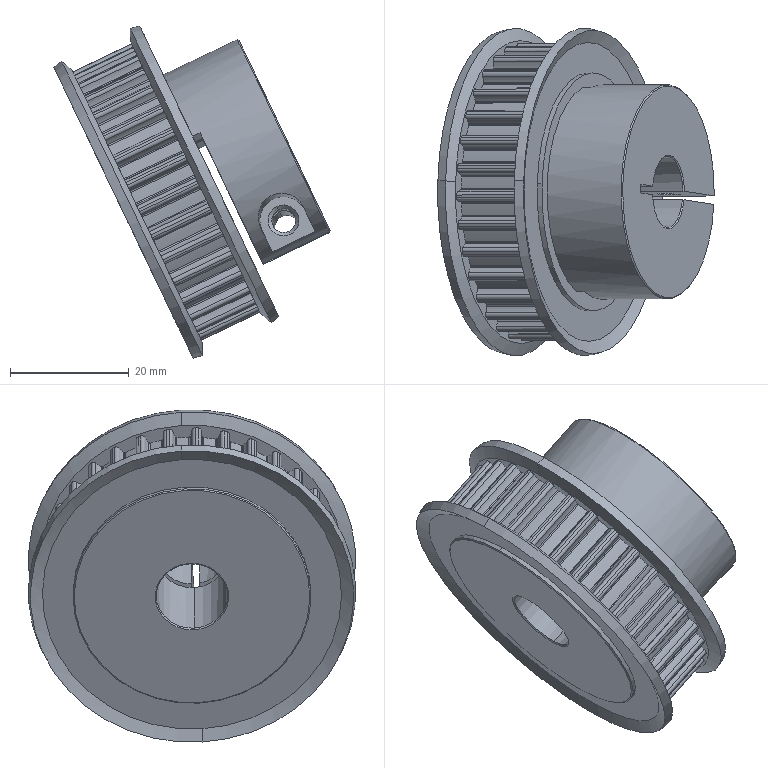Component | SolidWorks | HTCPA32_S5M100_12-1_HTCPA32_S5M100_12pulley-1 | 1 solid | 343 faces | volume 38720 mm3 | cylinder 301 | cone 22 | plane 20 | commonest cylinder face diameters 1.1 x80 0.5 x76 6.55 x68 46.43 x33 49.97 x32 4 x4 40 x4 12 x2